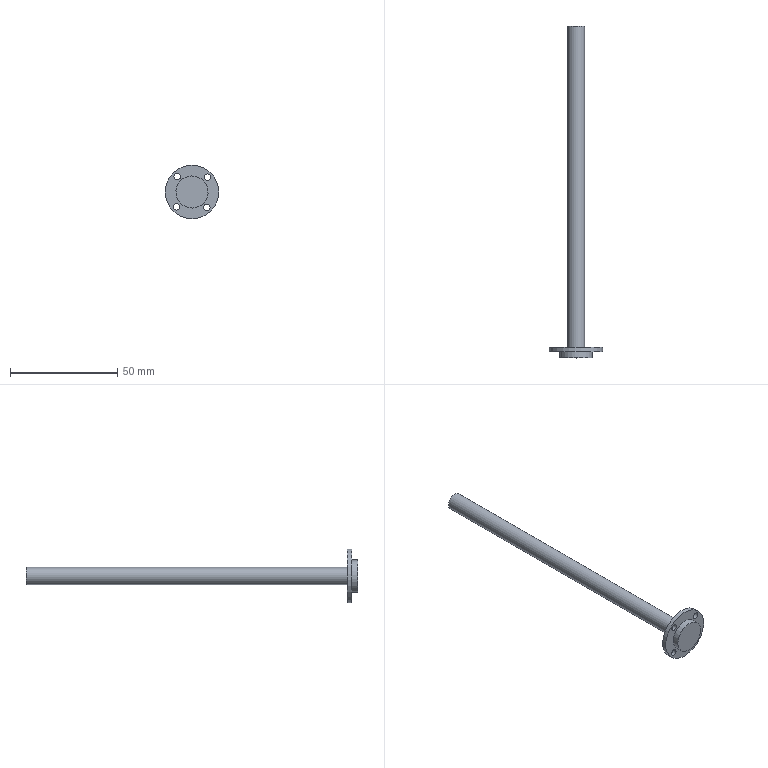Component | NX | GEAR_SHAFT_1 | 1 solid | 11 faces | box 25 x 155 x 25 mm | volume 8995 mm3 | cylinder 7 | plane 4 | commonest cylinder face diameters 3 x4 8 x1 25 x1 15 x1
STEP:
#1=CARTESIAN_POINT('',(0.,0.,0.));
#2=DIRECTION('',(0.,0.,1.));
#3=DIRECTION('',(1.,0.,0.));
#4=AXIS2_PLACEMENT_3D('',#1,#2,#3);
#5=CARTESIAN_POINT('',(-91.15,115.04,41.934));
#6=VERTEX_POINT('',#5);
#7=CARTESIAN_POINT('',(-88.383,115.04,39.046));
#8=DIRECTION('',(0.,-1.,0.));
#9=DIRECTION('',(-0.6919,0.,0.722));
#10=AXIS2_PLACEMENT_3D('',#7,#8,#9);
#11=CIRCLE('',#10,4.);
#12=CARTESIAN_POINT('',(-88.383,115.04,39.046));
#13=DIRECTION('',(0.,-1.,0.));
#14=DIRECTION('',(0.722,0.,0.6919));
#15=AXIS2_PLACEMENT_3D('',#12,#13,#14);
#16=CYLINDRICAL_SURFACE('',#15,4.);
#17=CARTESIAN_POINT('',(1.571,0.));
#18=DIRECTION('',(1.,0.));
#19=VECTOR('',#18,1.);
#20=LINE('',#17,#19);
#21=(GEOMETRIC_REPRESENTATION_CONTEXT(2)PARAMETRIC_REPRESENTATION_CONTEXT()REPRESENTATION_CONTEXT('',''));
#22=DEFINITIONAL_REPRESENTATION('',(#20),#21);
#23=PCURVE('',#16,#22);
#24=CARTESIAN_POINT('',(-88.383,115.04,39.046));
#25=DIRECTION('',(0.,-1.,0.));
#26=DIRECTION('',(0.722,0.,0.6919));
#27=AXIS2_PLACEMENT_3D('',#24,#25,#26);
#28=PLANE('',#27);
#29=CARTESIAN_POINT('',(0.,0.));
#30=DIRECTION('',(0.,1.));
#31=AXIS2_PLACEMENT_2D('',#29,#30);
#32=CIRCLE('',#31,4.);
#33=(GEOMETRIC_REPRESENTATION_CONTEXT(2)PARAMETRIC_REPRESENTATION_CONTEXT()REPRESENTATION_CONTEXT('',''));
#34=DEFINITIONAL_REPRESENTATION('',(#32),#33);
#35=PCURVE('',#28,#34);
#36=SURFACE_CURVE('',#11,(#23,#35),.PCURVE_S1.);
#37=EDGE_CURVE('',#6,#6,#36,.T.);
#38=ORIENTED_EDGE('',*,*,#37,.T.);
#39=CARTESIAN_POINT('',(-91.15,-34.96,41.934));
#40=VERTEX_POINT('',#39);
#41=CARTESIAN_POINT('',(-91.15,115.04,41.934));
#42=CARTESIAN_POINT('',(-91.15,-34.96,41.934));
#43=B_SPLINE_CURVE_WITH_KNOTS('',1,(#41,#42),.UNSPECIFIED.,.F.,.F.,(2,2),(0.,150.),.PIECEWISE_BEZIER_KNOTS.);
#44=CARTESIAN_POINT('',(7.854,0.));
#45=DIRECTION('',(0.,1.));
#46=VECTOR('',#45,1.);
#47=LINE('',#44,#46);
#48=(GEOMETRIC_REPRESENTATION_CONTEXT(2)PARAMETRIC_REPRESENTATION_CONTEXT()REPRESENTATION_CONTEXT('',''));
#49=DEFINITIONAL_REPRESENTATION('',(#47),#48);
#50=PCURVE('',#16,#49);
#51=CARTESIAN_POINT('',(1.571,0.));
#52=DIRECTION('',(0.,1.));
#53=VECTOR('',#52,1.);
#54=LINE('',#51,#53);
#55=(GEOMETRIC_REPRESENTATION_CONTEXT(2)PARAMETRIC_REPRESENTATION_CONTEXT()REPRESENTATION_CONTEXT('',''));
#56=DEFINITIONAL_REPRESENTATION('',(#54),#55);
#57=PCURVE('',#16,#56);
#58=SEAM_CURVE('',#43,(#50,#57),.PCURVE_S1.);
#59=EDGE_CURVE('',#6,#40,#58,.T.);
#60=ORIENTED_EDGE('',*,*,#59,.T.);
#61=CARTESIAN_POINT('',(-88.383,-34.96,39.046));
#62=DIRECTION('',(0.,-1.,0.));
#63=DIRECTION('',(-0.6919,0.,0.722));
#64=AXIS2_PLACEMENT_3D('',#61,#62,#63);
#65=CIRCLE('',#64,4.);
#66=CARTESIAN_POINT('',(1.571,150.));
#67=DIRECTION('',(1.,0.));
#68=VECTOR('',#67,1.);
#69=LINE('',#66,#68);
#70=(GEOMETRIC_REPRESENTATION_CONTEXT(2)PARAMETRIC_REPRESENTATION_CONTEXT()REPRESENTATION_CONTEXT('',''));
#71=DEFINITIONAL_REPRESENTATION('',(#69),#70);
#72=PCURVE('',#16,#71);
#73=CARTESIAN_POINT('',(-88.383,-34.96,39.046));
#74=DIRECTION('',(0.,-1.,0.));
#75=DIRECTION('',(0.722,0.,0.6919));
#76=AXIS2_PLACEMENT_3D('',#73,#74,#75);
#77=PLANE('',#76);
#78=CARTESIAN_POINT('',(0.,0.));
#79=DIRECTION('',(0.,1.));
#80=AXIS2_PLACEMENT_2D('',#78,#79);
#81=CIRCLE('',#80,4.);
#82=(GEOMETRIC_REPRESENTATION_CONTEXT(2)PARAMETRIC_REPRESENTATION_CONTEXT()REPRESENTATION_CONTEXT('',''));
#83=DEFINITIONAL_REPRESENTATION('',(#81),#82);
#84=PCURVE('',#77,#83);
#85=SURFACE_CURVE('',#65,(#72,#84),.PCURVE_S1.);
#86=EDGE_CURVE('',#40,#40,#85,.T.);
#87=ORIENTED_EDGE('',*,*,#86,.F.);
#88=ORIENTED_EDGE('',*,*,#59,.F.);
#89=EDGE_LOOP('',(#38,#60,#87,#88));
#90=FACE_BOUND('',#89,.T.);
#91=ADVANCED_FACE('',(#90),#16,.T.);
#92=ORIENTED_EDGE('',*,*,#37,.F.);
#93=EDGE_LOOP('',(#92));
#94=FACE_BOUND('',#93,.T.);
#95=ADVANCED_FACE('',(#94),#28,.F.);
#96=CARTESIAN_POINT('',(-97.032,-36.96,48.071));
#97=VERTEX_POINT('',#96);
#98=CARTESIAN_POINT('',(-88.383,-36.96,39.046));
#99=DIRECTION('',(0.,1.,0.));
#100=DIRECTION('',(-0.6919,0.,0.722));
#101=AXIS2_PLACEMENT_3D('',#98,#99,#100);
#102=CIRCLE('',#101,12.5);
#103=CARTESIAN_POINT('',(-88.383,-36.96,39.046));
#104=DIRECTION('',(0.,1.,0.));
#105=DIRECTION('',(-0.722,0.,-0.6919));
#106=AXIS2_PLACEMENT_3D('',#103,#104,#105);
#107=CYLINDRICAL_SURFACE('',#106,12.5);
#108=CARTESIAN_POINT('',(1.571,0.));
#109=DIRECTION('',(1.,0.));
#110=VECTOR('',#109,1.);
#111=LINE('',#108,#110);
#112=(GEOMETRIC_REPRESENTATION_CONTEXT(2)PARAMETRIC_REPRESENTATION_CONTEXT()REPRESENTATION_CONTEXT('',''));
#113=DEFINITIONAL_REPRESENTATION('',(#111),#112);
#114=PCURVE('',#107,#113);
#115=CARTESIAN_POINT('',(-88.383,-36.96,39.046));
#116=DIRECTION('',(0.,-1.,0.));
#117=DIRECTION('',(0.722,0.,0.6919));
#118=AXIS2_PLACEMENT_3D('',#115,#116,#117);
#119=PLANE('',#118);
#120=CARTESIAN_POINT('',(0.,12.5));
#121=CARTESIAN_POINT('',(21.651,12.5));
#122=CARTESIAN_POINT('',(10.825,-6.25));
#123=CARTESIAN_POINT('',(-0.,-25.));
#124=CARTESIAN_POINT('',(-10.825,-6.25));
#125=CARTESIAN_POINT('',(-21.651,12.5));
#126=CARTESIAN_POINT('',(0.,12.5));
#127=(BOUNDED_CURVE()B_SPLINE_CURVE(2,(#120,#121,#122,#123,#124,#125,#126),.UNSPECIFIED.,.T.,.F.)B_SPLINE_CURVE_WITH_KNOTS((1,2,2,2,2,1),(-2.094,0.,2.094,4.189,6.283,8.378),.UNSPECIFIED.)CURVE()GEOMETRIC_REPRESENTATION_ITEM()RATIONAL_B_SPLINE_CURVE((1.,0.5,1.,0.5,1.,0.5,1.))REPRESENTATION_ITEM(''));
#128=(GEOMETRIC_REPRESENTATION_CONTEXT(2)PARAMETRIC_REPRESENTATION_CONTEXT()REPRESENTATION_CONTEXT('',''));
#129=DEFINITIONAL_REPRESENTATION('',(#127),#128);
#130=PCURVE('',#119,#129);
#131=SURFACE_CURVE('',#102,(#114,#130),.PCURVE_S1.);
#132=EDGE_CURVE('',#97,#97,#131,.T.);
#133=ORIENTED_EDGE('',*,*,#132,.T.);
#134=CARTESIAN_POINT('',(-97.032,-34.96,48.071));
#135=VERTEX_POINT('',#134);
#136=CARTESIAN_POINT('',(-97.032,-36.96,48.071));
#137=CARTESIAN_POINT('',(-97.032,-34.96,48.071));
#138=B_SPLINE_CURVE_WITH_KNOTS('',1,(#136,#137),.UNSPECIFIED.,.F.,.F.,(2,2),(0.,2.),.PIECEWISE_BEZIER_KNOTS.);
#139=CARTESIAN_POINT('',(7.854,0.));
#140=DIRECTION('',(0.,1.));
#141=VECTOR('',#140,1.);
#142=LINE('',#139,#141);
#143=(GEOMETRIC_REPRESENTATION_CONTEXT(2)PARAMETRIC_REPRESENTATION_CONTEXT()REPRESENTATION_CONTEXT('',''));
#144=DEFINITIONAL_REPRESENTATION('',(#142),#143);
#145=PCURVE('',#107,#144);
#146=CARTESIAN_POINT('',(1.571,0.));
#147=DIRECTION('',(0.,1.));
#148=VECTOR('',#147,1.);
#149=LINE('',#146,#148);
#150=(GEOMETRIC_REPRESENTATION_CONTEXT(2)PARAMETRIC_REPRESENTATION_CONTEXT()REPRESENTATION_CONTEXT('',''));
#151=DEFINITIONAL_REPRESENTATION('',(#149),#150);
#152=PCURVE('',#107,#151);
#153=SEAM_CURVE('',#138,(#145,#152),.PCURVE_S1.);
#154=EDGE_CURVE('',#97,#135,#153,.T.);
#155=ORIENTED_EDGE('',*,*,#154,.T.);
#156=CARTESIAN_POINT('',(-88.383,-34.96,39.046));
#157=DIRECTION('',(0.,1.,0.));
#158=DIRECTION('',(-0.6919,0.,0.722));
#159=AXIS2_PLACEMENT_3D('',#156,#157,#158);
#160=CIRCLE('',#159,12.5);
#161=CARTESIAN_POINT('',(1.571,2.));
#162=DIRECTION('',(1.,0.));
#163=VECTOR('',#162,1.);
#164=LINE('',#161,#163);
#165=(GEOMETRIC_REPRESENTATION_CONTEXT(2)PARAMETRIC_REPRESENTATION_CONTEXT()REPRESENTATION_CONTEXT('',''));
#166=DEFINITIONAL_REPRESENTATION('',(#164),#165);
#167=PCURVE('',#107,#166);
#168=CARTESIAN_POINT('',(0.,12.5));
#169=CARTESIAN_POINT('',(21.651,12.5));
#170=CARTESIAN_POINT('',(10.825,-6.25));
#171=CARTESIAN_POINT('',(-0.,-25.));
#172=CARTESIAN_POINT('',(-10.825,-6.25));
#173=CARTESIAN_POINT('',(-21.651,12.5));
#174=CARTESIAN_POINT('',(0.,12.5));
#175=(BOUNDED_CURVE()B_SPLINE_CURVE(2,(#168,#169,#170,#171,#172,#173,#174),.UNSPECIFIED.,.T.,.F.)B_SPLINE_CURVE_WITH_KNOTS((1,2,2,2,2,1),(-2.094,0.,2.094,4.189,6.283,8.378),.UNSPECIFIED.)CURVE()GEOMETRIC_REPRESENTATION_ITEM()RATIONAL_B_SPLINE_CURVE((1.,0.5,1.,0.5,1.,0.5,1.))REPRESENTATION_ITEM(''));
#176=(GEOMETRIC_REPRESENTATION_CONTEXT(2)PARAMETRIC_REPRESENTATION_CONTEXT()REPRESENTATION_CONTEXT('',''));
#177=DEFINITIONAL_REPRESENTATION('',(#175),#176);
#178=PCURVE('',#77,#177);
#179=SURFACE_CURVE('',#160,(#167,#178),.PCURVE_S1.);
#180=EDGE_CURVE('',#135,#135,#179,.T.);
#181=ORIENTED_EDGE('',*,*,#180,.F.);
#182=ORIENTED_EDGE('',*,*,#154,.F.);
#183=EDGE_LOOP('',(#133,#155,#181,#182));
#184=FACE_BOUND('',#183,.T.);
#185=ADVANCED_FACE('',(#184),#107,.T.);
#186=CARTESIAN_POINT('',(-96.685,-36.96,31.089));
#187=VERTEX_POINT('',#186);
#188=CARTESIAN_POINT('',(-94.519,-36.96,33.165));
#189=VERTEX_POINT('',#188);
#190=CARTESIAN_POINT('',(-95.602,-36.96,32.127));
#191=DIRECTION('',(0.,1.,0.));
#192=DIRECTION('',(-0.722,0.,-0.6919));
#193=AXIS2_PLACEMENT_3D('',#190,#191,#192);
#194=CIRCLE('',#193,1.5);
#195=CARTESIAN_POINT('',(-11.5,0.));
#196=CARTESIAN_POINT('',(-11.5,2.598));
#197=CARTESIAN_POINT('',(-9.25,1.299));
#198=CARTESIAN_POINT('',(-7.,0.));
#199=CARTESIAN_POINT('',(-9.25,-1.299));
#200=CARTESIAN_POINT('',(-11.5,-2.598));
#201=CARTESIAN_POINT('',(-11.5,0.));
#202=(BOUNDED_CURVE()B_SPLINE_CURVE(2,(#195,#196,#197,#198,#199,#200,#201),.UNSPECIFIED.,.T.,.F.)B_SPLINE_CURVE_WITH_KNOTS((1,2,2,2,2,1),(-2.094,0.,2.094,4.189,6.283,8.378),.UNSPECIFIED.)CURVE()GEOMETRIC_REPRESENTATION_ITEM()RATIONAL_B_SPLINE_CURVE((1.,0.5,1.,0.5,1.,0.5,1.))REPRESENTATION_ITEM(''));
#203=(GEOMETRIC_REPRESENTATION_CONTEXT(2)PARAMETRIC_REPRESENTATION_CONTEXT()REPRESENTATION_CONTEXT('',''));
#204=DEFINITIONAL_REPRESENTATION('',(#202),#203);
#205=PCURVE('',#119,#204);
#206=CARTESIAN_POINT('',(-95.602,163.04,32.127));
#207=DIRECTION('',(0.,-1.,0.));
#208=DIRECTION('',(0.722,0.,0.6919));
#209=AXIS2_PLACEMENT_3D('',#206,#207,#208);
#210=CYLINDRICAL_SURFACE('',#209,1.5);
#211=CARTESIAN_POINT('',(3.142,200.));
#212=DIRECTION('',(-1.,0.));
#213=VECTOR('',#212,1.);
#214=LINE('',#211,#213);
#215=(GEOMETRIC_REPRESENTATION_CONTEXT(2)PARAMETRIC_REPRESENTATION_CONTEXT()REPRESENTATION_CONTEXT('',''));
#216=DEFINITIONAL_REPRESENTATION('',(#214),#215);
#217=PCURVE('',#210,#216);
#218=SURFACE_CURVE('',#194,(#205,#217),.PCURVE_S1.);
#219=EDGE_CURVE('',#187,#189,#218,.T.);
#220=ORIENTED_EDGE('',*,*,#219,.T.);
#221=CARTESIAN_POINT('',(-95.602,-36.96,32.127));
#222=DIRECTION('',(0.,1.,0.));
#223=DIRECTION('',(-0.722,0.,-0.6919));
#224=AXIS2_PLACEMENT_3D('',#221,#222,#223);
#225=CIRCLE('',#224,1.5);
#226=CARTESIAN_POINT('',(-11.5,0.));
#227=CARTESIAN_POINT('',(-11.5,2.598));
#228=CARTESIAN_POINT('',(-9.25,1.299));
#229=CARTESIAN_POINT('',(-7.,0.));
#230=CARTESIAN_POINT('',(-9.25,-1.299));
#231=CARTESIAN_POINT('',(-11.5,-2.598));
#232=CARTESIAN_POINT('',(-11.5,0.));
#233=(BOUNDED_CURVE()B_SPLINE_CURVE(2,(#226,#227,#228,#229,#230,#231,#232),.UNSPECIFIED.,.T.,.F.)B_SPLINE_CURVE_WITH_KNOTS((1,2,2,2,2,1),(-2.094,0.,2.094,4.189,6.283,8.378),.UNSPECIFIED.)CURVE()GEOMETRIC_REPRESENTATION_ITEM()RATIONAL_B_SPLINE_CURVE((1.,0.5,1.,0.5,1.,0.5,1.))REPRESENTATION_ITEM(''));
#234=(GEOMETRIC_REPRESENTATION_CONTEXT(2)PARAMETRIC_REPRESENTATION_CONTEXT()REPRESENTATION_CONTEXT('',''));
#235=DEFINITIONAL_REPRESENTATION('',(#233),#234);
#236=PCURVE('',#119,#235);
#237=CARTESIAN_POINT('',(9.425,200.));
#238=DIRECTION('',(-1.,0.));
#239=VECTOR('',#238,1.);
#240=LINE('',#237,#239);
#241=(GEOMETRIC_REPRESENTATION_CONTEXT(2)PARAMETRIC_REPRESENTATION_CONTEXT()REPRESENTATION_CONTEXT('',''));
#242=DEFINITIONAL_REPRESENTATION('',(#240),#241);
#243=PCURVE('',#210,#242);
#244=SURFACE_CURVE('',#225,(#236,#243),.PCURVE_S1.);
#245=EDGE_CURVE('',#189,#187,#244,.T.);
#246=ORIENTED_EDGE('',*,*,#245,.T.);
#247=EDGE_LOOP('',(#220,#246));
#248=FACE_BOUND('',#247,.T.);
#249=CARTESIAN_POINT('',(-80.426,-36.96,30.744));
#250=VERTEX_POINT('',#249);
#251=CARTESIAN_POINT('',(-80.381,-36.96,32.865));
#252=VERTEX_POINT('',#251);
#253=CARTESIAN_POINT('',(-81.463,-36.96,31.827));
#254=DIRECTION('',(0.,-1.,0.));
#255=DIRECTION('',(0.6919,0.,-0.722));
#256=AXIS2_PLACEMENT_3D('',#253,#254,#255);
#257=CIRCLE('',#256,1.5);
#258=CARTESIAN_POINT('',(-0.,-10.));
#259=DIRECTION('',(-0.,-1.));
#260=AXIS2_PLACEMENT_2D('',#258,#259);
#261=CIRCLE('',#260,1.5);
#262=(GEOMETRIC_REPRESENTATION_CONTEXT(2)PARAMETRIC_REPRESENTATION_CONTEXT()REPRESENTATION_CONTEXT('',''));
#263=DEFINITIONAL_REPRESENTATION('',(#261),#262);
#264=PCURVE('',#119,#263);
#265=CARTESIAN_POINT('',(-81.463,163.04,31.827));
#266=DIRECTION('',(0.,-1.,0.));
#267=DIRECTION('',(0.722,0.,0.6919));
#268=AXIS2_PLACEMENT_3D('',#265,#266,#267);
#269=CYLINDRICAL_SURFACE('',#268,1.5);
#270=CARTESIAN_POINT('',(4.712,200.));
#271=DIRECTION('',(1.,0.));
#272=VECTOR('',#271,1.);
#273=LINE('',#270,#272);
#274=(GEOMETRIC_REPRESENTATION_CONTEXT(2)PARAMETRIC_REPRESENTATION_CONTEXT()REPRESENTATION_CONTEXT('',''));
#275=DEFINITIONAL_REPRESENTATION('',(#273),#274);
#276=PCURVE('',#269,#275);
#277=SURFACE_CURVE('',#257,(#264,#276),.PCURVE_S1.);
#278=EDGE_CURVE('',#250,#252,#277,.T.);
#279=ORIENTED_EDGE('',*,*,#278,.F.);
#280=CARTESIAN_POINT('',(-81.463,-36.96,31.827));
#281=DIRECTION('',(0.,-1.,0.));
#282=DIRECTION('',(0.6919,0.,-0.722));
#283=AXIS2_PLACEMENT_3D('',#280,#281,#282);
#284=CIRCLE('',#283,1.5);
#285=CARTESIAN_POINT('',(-0.,-10.));
#286=DIRECTION('',(-0.,-1.));
#287=AXIS2_PLACEMENT_2D('',#285,#286);
#288=CIRCLE('',#287,1.5);
#289=(GEOMETRIC_REPRESENTATION_CONTEXT(2)PARAMETRIC_REPRESENTATION_CONTEXT()REPRESENTATION_CONTEXT('',''));
#290=DEFINITIONAL_REPRESENTATION('',(#288),#289);
#291=PCURVE('',#119,#290);
#292=CARTESIAN_POINT('',(-1.571,200.));
#293=DIRECTION('',(1.,0.));
#294=VECTOR('',#293,1.);
#295=LINE('',#292,#294);
#296=(GEOMETRIC_REPRESENTATION_CONTEXT(2)PARAMETRIC_REPRESENTATION_CONTEXT()REPRESENTATION_CONTEXT('',''));
#297=DEFINITIONAL_REPRESENTATION('',(#295),#296);
#298=PCURVE('',#269,#297);
#299=SURFACE_CURVE('',#284,(#291,#298),.PCURVE_S1.);
#300=EDGE_CURVE('',#252,#250,#299,.T.);
#301=ORIENTED_EDGE('',*,*,#300,.F.);
#302=EDGE_LOOP('',(#279,#301));
#303=FACE_BOUND('',#302,.T.);
#304=CARTESIAN_POINT('',(-80.08,-36.96,47.004));
#305=VERTEX_POINT('',#304);
#306=CARTESIAN_POINT('',(-81.163,-36.96,45.966));
#307=DIRECTION('',(0.,-1.,0.));
#308=DIRECTION('',(0.722,0.,0.6919));
#309=AXIS2_PLACEMENT_3D('',#306,#307,#308);
#310=CIRCLE('',#309,1.5);
#311=CARTESIAN_POINT('',(10.,0.));
#312=DIRECTION('',(1.,-0.));
#313=AXIS2_PLACEMENT_2D('',#311,#312);
#314=CIRCLE('',#313,1.5);
#315=(GEOMETRIC_REPRESENTATION_CONTEXT(2)PARAMETRIC_REPRESENTATION_CONTEXT()REPRESENTATION_CONTEXT('',''));
#316=DEFINITIONAL_REPRESENTATION('',(#314),#315);
#317=PCURVE('',#119,#316);
#318=CARTESIAN_POINT('',(-81.163,163.04,45.966));
#319=DIRECTION('',(0.,-1.,0.));
#320=DIRECTION('',(0.722,0.,0.6919));
#321=AXIS2_PLACEMENT_3D('',#318,#319,#320);
#322=CYLINDRICAL_SURFACE('',#321,1.5);
#323=CARTESIAN_POINT('',(0.,200.));
#324=DIRECTION('',(1.,0.));
#325=VECTOR('',#324,1.);
#326=LINE('',#323,#325);
#327=(GEOMETRIC_REPRESENTATION_CONTEXT(2)PARAMETRIC_REPRESENTATION_CONTEXT()REPRESENTATION_CONTEXT('',''));
#328=DEFINITIONAL_REPRESENTATION('',(#326),#327);
#329=PCURVE('',#322,#328);
#330=SURFACE_CURVE('',#310,(#317,#329),.PCURVE_S1.);
#331=EDGE_CURVE('',#305,#305,#330,.T.);
#332=ORIENTED_EDGE('',*,*,#331,.F.);
#333=EDGE_LOOP('',(#332));
#334=FACE_BOUND('',#333,.T.);
#335=CARTESIAN_POINT('',(-96.34,-36.96,47.349));
#336=VERTEX_POINT('',#335);
#337=CARTESIAN_POINT('',(-94.219,-36.96,47.304));
#338=VERTEX_POINT('',#337);
#339=CARTESIAN_POINT('',(-95.302,-36.96,46.266));
#340=DIRECTION('',(0.,-1.,0.));
#341=DIRECTION('',(-0.6919,0.,0.722));
#342=AXIS2_PLACEMENT_3D('',#339,#340,#341);
#343=CIRCLE('',#342,1.5);
#344=CARTESIAN_POINT('',(-0.,10.));
#345=DIRECTION('',(0.,1.));
#346=AXIS2_PLACEMENT_2D('',#344,#345);
#347=CIRCLE('',#346,1.5);
#348=(GEOMETRIC_REPRESENTATION_CONTEXT(2)PARAMETRIC_REPRESENTATION_CONTEXT()REPRESENTATION_CONTEXT('',''));
#349=DEFINITIONAL_REPRESENTATION('',(#347),#348);
#350=PCURVE('',#119,#349);
#351=CARTESIAN_POINT('',(-95.302,163.04,46.266));
#352=DIRECTION('',(0.,-1.,0.));
#353=DIRECTION('',(0.722,0.,0.6919));
#354=AXIS2_PLACEMENT_3D('',#351,#352,#353);
#355=CYLINDRICAL_SURFACE('',#354,1.5);
#356=CARTESIAN_POINT('',(1.571,200.));
#357=DIRECTION('',(1.,0.));
#358=VECTOR('',#357,1.);
#359=LINE('',#356,#358);
#360=(GEOMETRIC_REPRESENTATION_CONTEXT(2)PARAMETRIC_REPRESENTATION_CONTEXT()REPRESENTATION_CONTEXT('',''));
#361=DEFINITIONAL_REPRESENTATION('',(#359),#360);
#362=PCURVE('',#355,#361);
#363=SURFACE_CURVE('',#343,(#350,#362),.PCURVE_S1.);
#364=EDGE_CURVE('',#336,#338,#363,.T.);
#365=ORIENTED_EDGE('',*,*,#364,.F.);
#366=CARTESIAN_POINT('',(-95.302,-36.96,46.266));
#367=DIRECTION('',(0.,-1.,0.));
#368=DIRECTION('',(-0.6919,0.,0.722));
#369=AXIS2_PLACEMENT_3D('',#366,#367,#368);
#370=CIRCLE('',#369,1.5);
#371=CARTESIAN_POINT('',(-0.,10.));
#372=DIRECTION('',(0.,1.));
#373=AXIS2_PLACEMENT_2D('',#371,#372);
#374=CIRCLE('',#373,1.5);
#375=(GEOMETRIC_REPRESENTATION_CONTEXT(2)PARAMETRIC_REPRESENTATION_CONTEXT()REPRESENTATION_CONTEXT('',''));
#376=DEFINITIONAL_REPRESENTATION('',(#374),#375);
#377=PCURVE('',#119,#376);
#378=CARTESIAN_POINT('',(-4.712,200.));
#379=DIRECTION('',(1.,0.));
#380=VECTOR('',#379,1.);
#381=LINE('',#378,#380);
#382=(GEOMETRIC_REPRESENTATION_CONTEXT(2)PARAMETRIC_REPRESENTATION_CONTEXT()REPRESENTATION_CONTEXT('',''));
#383=DEFINITIONAL_REPRESENTATION('',(#381),#382);
#384=PCURVE('',#355,#383);
#385=SURFACE_CURVE('',#370,(#377,#384),.PCURVE_S1.);
#386=EDGE_CURVE('',#338,#336,#385,.T.);
#387=ORIENTED_EDGE('',*,*,#386,.F.);
#388=EDGE_LOOP('',(#365,#387));
#389=FACE_BOUND('',#388,.T.);
#390=CARTESIAN_POINT('',(-93.572,-36.96,44.461));
#391=VERTEX_POINT('',#390);
#392=CARTESIAN_POINT('',(-88.383,-36.96,39.046));
#393=DIRECTION('',(0.,-1.,0.));
#394=DIRECTION('',(-0.6919,0.,0.722));
#395=AXIS2_PLACEMENT_3D('',#392,#393,#394);
#396=CIRCLE('',#395,7.5);
#397=CARTESIAN_POINT('',(0.,0.));
#398=DIRECTION('',(0.,1.));
#399=AXIS2_PLACEMENT_2D('',#397,#398);
#400=CIRCLE('',#399,7.5);
#401=(GEOMETRIC_REPRESENTATION_CONTEXT(2)PARAMETRIC_REPRESENTATION_CONTEXT()REPRESENTATION_CONTEXT('',''));
#402=DEFINITIONAL_REPRESENTATION('',(#400),#401);
#403=PCURVE('',#119,#402);
#404=CARTESIAN_POINT('',(-88.383,-39.96,39.046));
#405=DIRECTION('',(0.,1.,0.));
#406=DIRECTION('',(-0.722,0.,-0.6919));
#407=AXIS2_PLACEMENT_3D('',#404,#405,#406);
#408=CYLINDRICAL_SURFACE('',#407,7.5);
#409=CARTESIAN_POINT('',(7.854,3.));
#410=DIRECTION('',(-1.,0.));
#411=VECTOR('',#410,1.);
#412=LINE('',#409,#411);
#413=(GEOMETRIC_REPRESENTATION_CONTEXT(2)PARAMETRIC_REPRESENTATION_CONTEXT()REPRESENTATION_CONTEXT('',''));
#414=DEFINITIONAL_REPRESENTATION('',(#412),#413);
#415=PCURVE('',#408,#414);
#416=SURFACE_CURVE('',#396,(#403,#415),.PCURVE_S1.);
#417=EDGE_CURVE('',#391,#391,#416,.T.);
#418=ORIENTED_EDGE('',*,*,#417,.F.);
#419=EDGE_LOOP('',(#418));
#420=FACE_BOUND('',#419,.T.);
#421=ORIENTED_EDGE('',*,*,#132,.F.);
#422=EDGE_LOOP('',(#421));
#423=FACE_BOUND('',#422,.T.);
#424=ADVANCED_FACE('',(#248,#303,#334,#389,#420,#423),#119,.T.);
#425=CARTESIAN_POINT('',(-94.519,-34.96,33.165));
#426=VERTEX_POINT('',#425);
#427=CARTESIAN_POINT('',(-95.602,-34.96,32.127));
#428=DIRECTION('',(0.,1.,0.));
#429=DIRECTION('',(0.722,0.,0.6919));
#430=AXIS2_PLACEMENT_3D('',#427,#428,#429);
#431=CIRCLE('',#430,1.5);
#432=CARTESIAN_POINT('',(-8.5,0.));
#433=CARTESIAN_POINT('',(-8.5,-2.598));
#434=CARTESIAN_POINT('',(-10.75,-1.299));
#435=CARTESIAN_POINT('',(-13.,0.));
#436=CARTESIAN_POINT('',(-10.75,1.299));
#437=CARTESIAN_POINT('',(-8.5,2.598));
#438=CARTESIAN_POINT('',(-8.5,0.));
#439=(BOUNDED_CURVE()B_SPLINE_CURVE(2,(#432,#433,#434,#435,#436,#437,#438),.UNSPECIFIED.,.T.,.F.)B_SPLINE_CURVE_WITH_KNOTS((1,2,2,2,2,1),(-2.094,0.,2.094,4.189,6.283,8.378),.UNSPECIFIED.)CURVE()GEOMETRIC_REPRESENTATION_ITEM()RATIONAL_B_SPLINE_CURVE((1.,0.5,1.,0.5,1.,0.5,1.))REPRESENTATION_ITEM(''));
#440=(GEOMETRIC_REPRESENTATION_CONTEXT(2)PARAMETRIC_REPRESENTATION_CONTEXT()REPRESENTATION_CONTEXT('',''));
#441=DEFINITIONAL_REPRESENTATION('',(#439),#440);
#442=PCURVE('',#77,#441);
#443=CARTESIAN_POINT('',(6.283,198.));
#444=DIRECTION('',(-1.,0.));
#445=VECTOR('',#444,1.);
#446=LINE('',#443,#445);
#447=(GEOMETRIC_REPRESENTATION_CONTEXT(2)PARAMETRIC_REPRESENTATION_CONTEXT()REPRESENTATION_CONTEXT('',''));
#448=DEFINITIONAL_REPRESENTATION('',(#446),#447);
#449=PCURVE('',#210,#448);
#450=SURFACE_CURVE('',#431,(#442,#449),.PCURVE_S1.);
#451=EDGE_CURVE('',#426,#426,#450,.T.);
#452=ORIENTED_EDGE('',*,*,#451,.F.);
#453=EDGE_LOOP('',(#452));
#454=FACE_BOUND('',#453,.T.);
#455=CARTESIAN_POINT('',(-80.381,-34.96,32.865));
#456=VERTEX_POINT('',#455);
#457=CARTESIAN_POINT('',(-81.463,-34.96,31.827));
#458=DIRECTION('',(0.,-1.,0.));
#459=DIRECTION('',(0.722,0.,0.6919));
#460=AXIS2_PLACEMENT_3D('',#457,#458,#459);
#461=CIRCLE('',#460,1.5);
#462=CARTESIAN_POINT('',(-0.,-10.));
#463=DIRECTION('',(1.,-0.));
#464=AXIS2_PLACEMENT_2D('',#462,#463);
#465=CIRCLE('',#464,1.5);
#466=(GEOMETRIC_REPRESENTATION_CONTEXT(2)PARAMETRIC_REPRESENTATION_CONTEXT()REPRESENTATION_CONTEXT('',''));
#467=DEFINITIONAL_REPRESENTATION('',(#465),#466);
#468=PCURVE('',#77,#467);
#469=CARTESIAN_POINT('',(0.,198.));
#470=DIRECTION('',(1.,0.));
#471=VECTOR('',#470,1.);
#472=LINE('',#469,#471);
#473=(GEOMETRIC_REPRESENTATION_CONTEXT(2)PARAMETRIC_REPRESENTATION_CONTEXT()REPRESENTATION_CONTEXT('',''));
#474=DEFINITIONAL_REPRESENTATION('',(#472),#473);
#475=PCURVE('',#269,#474);
#476=SURFACE_CURVE('',#461,(#468,#475),.PCURVE_S1.);
#477=EDGE_CURVE('',#456,#456,#476,.T.);
#478=ORIENTED_EDGE('',*,*,#477,.T.);
#479=EDGE_LOOP('',(#478));
#480=FACE_BOUND('',#479,.T.);
#481=CARTESIAN_POINT('',(-80.08,-34.96,47.004));
#482=VERTEX_POINT('',#481);
#483=CARTESIAN_POINT('',(-81.163,-34.96,45.966));
#484=DIRECTION('',(0.,-1.,0.));
#485=DIRECTION('',(0.722,0.,0.6919));
#486=AXIS2_PLACEMENT_3D('',#483,#484,#485);
#487=CIRCLE('',#486,1.5);
#488=CARTESIAN_POINT('',(10.,0.));
#489=DIRECTION('',(1.,-0.));
#490=AXIS2_PLACEMENT_2D('',#488,#489);
#491=CIRCLE('',#490,1.5);
#492=(GEOMETRIC_REPRESENTATION_CONTEXT(2)PARAMETRIC_REPRESENTATION_CONTEXT()REPRESENTATION_CONTEXT('',''));
#493=DEFINITIONAL_REPRESENTATION('',(#491),#492);
#494=PCURVE('',#77,#493);
#495=CARTESIAN_POINT('',(0.,198.));
#496=DIRECTION('',(1.,0.));
#497=VECTOR('',#496,1.);
#498=LINE('',#495,#497);
#499=(GEOMETRIC_REPRESENTATION_CONTEXT(2)PARAMETRIC_REPRESENTATION_CONTEXT()REPRESENTATION_CONTEXT('',''));
#500=DEFINITIONAL_REPRESENTATION('',(#498),#499);
#501=PCURVE('',#322,#500);
#502=SURFACE_CURVE('',#487,(#494,#501),.PCURVE_S1.);
#503=EDGE_CURVE('',#482,#482,#502,.T.);
#504=ORIENTED_EDGE('',*,*,#503,.T.);
#505=EDGE_LOOP('',(#504));
#506=FACE_BOUND('',#505,.T.);
#507=CARTESIAN_POINT('',(-94.219,-34.96,47.304));
#508=VERTEX_POINT('',#507);
#509=CARTESIAN_POINT('',(-95.302,-34.96,46.266));
#510=DIRECTION('',(0.,-1.,0.));
#511=DIRECTION('',(0.722,0.,0.6919));
#512=AXIS2_PLACEMENT_3D('',#509,#510,#511);
#513=CIRCLE('',#512,1.5);
#514=CARTESIAN_POINT('',(-0.,10.));
#515=DIRECTION('',(1.,-0.));
#516=AXIS2_PLACEMENT_2D('',#514,#515);
#517=CIRCLE('',#516,1.5);
#518=(GEOMETRIC_REPRESENTATION_CONTEXT(2)PARAMETRIC_REPRESENTATION_CONTEXT()REPRESENTATION_CONTEXT('',''));
#519=DEFINITIONAL_REPRESENTATION('',(#517),#518);
#520=PCURVE('',#77,#519);
#521=CARTESIAN_POINT('',(0.,198.));
#522=DIRECTION('',(1.,0.));
#523=VECTOR('',#522,1.);
#524=LINE('',#521,#523);
#525=(GEOMETRIC_REPRESENTATION_CONTEXT(2)PARAMETRIC_REPRESENTATION_CONTEXT()REPRESENTATION_CONTEXT('',''));
#526=DEFINITIONAL_REPRESENTATION('',(#524),#525);
#527=PCURVE('',#355,#526);
#528=SURFACE_CURVE('',#513,(#520,#527),.PCURVE_S1.);
#529=EDGE_CURVE('',#508,#508,#528,.T.);
#530=ORIENTED_EDGE('',*,*,#529,.T.);
#531=EDGE_LOOP('',(#530));
#532=FACE_BOUND('',#531,.T.);
#533=ORIENTED_EDGE('',*,*,#86,.T.);
#534=EDGE_LOOP('',(#533));
#535=FACE_BOUND('',#534,.T.);
#536=ORIENTED_EDGE('',*,*,#180,.T.);
#537=EDGE_LOOP('',(#536));
#538=FACE_BOUND('',#537,.T.);
#539=ADVANCED_FACE('',(#454,#480,#506,#532,#535,#538),#77,.F.);
#540=CARTESIAN_POINT('',(-93.572,-39.96,44.461));
#541=VERTEX_POINT('',#540);
#542=CARTESIAN_POINT('',(-88.383,-39.96,39.046));
#543=DIRECTION('',(0.,-1.,0.));
#544=DIRECTION('',(-0.6919,0.,0.722));
#545=AXIS2_PLACEMENT_3D('',#542,#543,#544);
#546=CIRCLE('',#545,7.5);
#547=CARTESIAN_POINT('',(7.854,0.));
#548=DIRECTION('',(-1.,0.));
#549=VECTOR('',#548,1.);
#550=LINE('',#547,#549);
#551=(GEOMETRIC_REPRESENTATION_CONTEXT(2)PARAMETRIC_REPRESENTATION_CONTEXT()REPRESENTATION_CONTEXT('',''));
#552=DEFINITIONAL_REPRESENTATION('',(#550),#551);
#553=PCURVE('',#408,#552);
#554=CARTESIAN_POINT('',(-88.383,-39.96,39.046));
#555=DIRECTION('',(0.,-1.,0.));
#556=DIRECTION('',(0.722,0.,0.6919));
#557=AXIS2_PLACEMENT_3D('',#554,#555,#556);
#558=PLANE('',#557);
#559=CARTESIAN_POINT('',(0.,0.));
#560=DIRECTION('',(0.,1.));
#561=AXIS2_PLACEMENT_2D('',#559,#560);
#562=CIRCLE('',#561,7.5);
#563=(GEOMETRIC_REPRESENTATION_CONTEXT(2)PARAMETRIC_REPRESENTATION_CONTEXT()REPRESENTATION_CONTEXT('',''));
#564=DEFINITIONAL_REPRESENTATION('',(#562),#563);
#565=PCURVE('',#558,#564);
#566=SURFACE_CURVE('',#546,(#553,#565),.PCURVE_S1.);
#567=EDGE_CURVE('',#541,#541,#566,.T.);
#568=ORIENTED_EDGE('',*,*,#567,.F.);
#569=CARTESIAN_POINT('',(-93.572,-39.96,44.461));
#570=CARTESIAN_POINT('',(-93.572,-36.96,44.461));
#571=B_SPLINE_CURVE_WITH_KNOTS('',1,(#569,#570),.UNSPECIFIED.,.F.,.F.,(2,2),(0.,3.),.PIECEWISE_BEZIER_KNOTS.);
#572=CARTESIAN_POINT('',(7.854,0.));
#573=DIRECTION('',(0.,1.));
#574=VECTOR('',#573,1.);
#575=LINE('',#572,#574);
#576=(GEOMETRIC_REPRESENTATION_CONTEXT(2)PARAMETRIC_REPRESENTATION_CONTEXT()REPRESENTATION_CONTEXT('',''));
#577=DEFINITIONAL_REPRESENTATION('',(#575),#576);
#578=PCURVE('',#408,#577);
#579=CARTESIAN_POINT('',(1.571,0.));
#580=DIRECTION('',(0.,1.));
#581=VECTOR('',#580,1.);
#582=LINE('',#579,#581);
#583=(GEOMETRIC_REPRESENTATION_CONTEXT(2)PARAMETRIC_REPRESENTATION_CONTEXT()REPRESENTATION_CONTEXT('',''));
#584=DEFINITIONAL_REPRESENTATION('',(#582),#583);
#585=PCURVE('',#408,#584);
#586=SEAM_CURVE('',#571,(#578,#585),.PCURVE_S1.);
#587=EDGE_CURVE('',#541,#391,#586,.T.);
#588=ORIENTED_EDGE('',*,*,#587,.T.);
#589=ORIENTED_EDGE('',*,*,#417,.T.);
#590=ORIENTED_EDGE('',*,*,#587,.F.);
#591=EDGE_LOOP('',(#568,#588,#589,#590));
#592=FACE_BOUND('',#591,.T.);
#593=ADVANCED_FACE('',(#592),#408,.T.);
#594=ORIENTED_EDGE('',*,*,#567,.T.);
#595=EDGE_LOOP('',(#594));
#596=FACE_BOUND('',#595,.T.);
#597=ADVANCED_FACE('',(#596),#558,.T.);
#598=ORIENTED_EDGE('',*,*,#386,.F.);
#599=CARTESIAN_POINT('',(-94.219,-34.96,47.304));
#600=CARTESIAN_POINT('',(-94.219,-36.96,47.304));
#601=B_SPLINE_CURVE_WITH_KNOTS('',1,(#599,#600),.UNSPECIFIED.,.F.,.F.,(2,2),(198.,200.),.PIECEWISE_BEZIER_KNOTS.);
#602=CARTESIAN_POINT('',(0.,0.));
#603=DIRECTION('',(0.,1.));
#604=VECTOR('',#603,1.);
#605=LINE('',#602,#604);
#606=(GEOMETRIC_REPRESENTATION_CONTEXT(2)PARAMETRIC_REPRESENTATION_CONTEXT()REPRESENTATION_CONTEXT('',''));
#607=DEFINITIONAL_REPRESENTATION('',(#605),#606);
#608=PCURVE('',#355,#607);
#609=CARTESIAN_POINT('',(6.283,0.));
#610=DIRECTION('',(0.,1.));
#611=VECTOR('',#610,1.);
#612=LINE('',#609,#611);
#613=(GEOMETRIC_REPRESENTATION_CONTEXT(2)PARAMETRIC_REPRESENTATION_CONTEXT()REPRESENTATION_CONTEXT('',''));
#614=DEFINITIONAL_REPRESENTATION('',(#612),#613);
#615=PCURVE('',#355,#614);
#616=SEAM_CURVE('',#601,(#608,#615),.PCURVE_S1.);
#617=EDGE_CURVE('',#508,#338,#616,.T.);
#618=ORIENTED_EDGE('',*,*,#617,.F.);
#619=ORIENTED_EDGE('',*,*,#529,.T.);
#620=ORIENTED_EDGE('',*,*,#617,.T.);
#621=ORIENTED_EDGE('',*,*,#364,.F.);
#622=EDGE_LOOP('',(#598,#618,#619,#620,#621));
#623=FACE_BOUND('',#622,.F.);
#624=ADVANCED_FACE('',(#623),#355,.F.);
#625=ORIENTED_EDGE('',*,*,#331,.F.);
#626=CARTESIAN_POINT('',(-80.08,-34.96,47.004));
#627=CARTESIAN_POINT('',(-80.08,-36.96,47.004));
#628=B_SPLINE_CURVE_WITH_KNOTS('',1,(#626,#627),.UNSPECIFIED.,.F.,.F.,(2,2),(198.,200.),.PIECEWISE_BEZIER_KNOTS.);
#629=CARTESIAN_POINT('',(0.,0.));
#630=DIRECTION('',(0.,1.));
#631=VECTOR('',#630,1.);
#632=LINE('',#629,#631);
#633=(GEOMETRIC_REPRESENTATION_CONTEXT(2)PARAMETRIC_REPRESENTATION_CONTEXT()REPRESENTATION_CONTEXT('',''));
#634=DEFINITIONAL_REPRESENTATION('',(#632),#633);
#635=PCURVE('',#322,#634);
#636=CARTESIAN_POINT('',(6.283,0.));
#637=DIRECTION('',(0.,1.));
#638=VECTOR('',#637,1.);
#639=LINE('',#636,#638);
#640=(GEOMETRIC_REPRESENTATION_CONTEXT(2)PARAMETRIC_REPRESENTATION_CONTEXT()REPRESENTATION_CONTEXT('',''));
#641=DEFINITIONAL_REPRESENTATION('',(#639),#640);
#642=PCURVE('',#322,#641);
#643=SEAM_CURVE('',#628,(#635,#642),.PCURVE_S1.);
#644=EDGE_CURVE('',#482,#305,#643,.T.);
#645=ORIENTED_EDGE('',*,*,#644,.F.);
#646=ORIENTED_EDGE('',*,*,#503,.T.);
#647=ORIENTED_EDGE('',*,*,#644,.T.);
#648=EDGE_LOOP('',(#625,#645,#646,#647));
#649=FACE_BOUND('',#648,.F.);
#650=ADVANCED_FACE('',(#649),#322,.F.);
#651=ORIENTED_EDGE('',*,*,#300,.F.);
#652=CARTESIAN_POINT('',(-80.381,-34.96,32.865));
#653=CARTESIAN_POINT('',(-80.381,-36.96,32.865));
#654=B_SPLINE_CURVE_WITH_KNOTS('',1,(#652,#653),.UNSPECIFIED.,.F.,.F.,(2,2),(198.,200.),.PIECEWISE_BEZIER_KNOTS.);
#655=CARTESIAN_POINT('',(0.,0.));
#656=DIRECTION('',(0.,1.));
#657=VECTOR('',#656,1.);
#658=LINE('',#655,#657);
#659=(GEOMETRIC_REPRESENTATION_CONTEXT(2)PARAMETRIC_REPRESENTATION_CONTEXT()REPRESENTATION_CONTEXT('',''));
#660=DEFINITIONAL_REPRESENTATION('',(#658),#659);
#661=PCURVE('',#269,#660);
#662=CARTESIAN_POINT('',(6.283,0.));
#663=DIRECTION('',(0.,1.));
#664=VECTOR('',#663,1.);
#665=LINE('',#662,#664);
#666=(GEOMETRIC_REPRESENTATION_CONTEXT(2)PARAMETRIC_REPRESENTATION_CONTEXT()REPRESENTATION_CONTEXT('',''));
#667=DEFINITIONAL_REPRESENTATION('',(#665),#666);
#668=PCURVE('',#269,#667);
#669=SEAM_CURVE('',#654,(#661,#668),.PCURVE_S1.);
#670=EDGE_CURVE('',#456,#252,#669,.T.);
#671=ORIENTED_EDGE('',*,*,#670,.F.);
#672=ORIENTED_EDGE('',*,*,#477,.T.);
#673=ORIENTED_EDGE('',*,*,#670,.T.);
#674=ORIENTED_EDGE('',*,*,#278,.F.);
#675=EDGE_LOOP('',(#651,#671,#672,#673,#674));
#676=FACE_BOUND('',#675,.F.);
#677=ADVANCED_FACE('',(#676),#269,.F.);
#678=ORIENTED_EDGE('',*,*,#219,.T.);
#679=CARTESIAN_POINT('',(-94.519,-34.96,33.165));
#680=CARTESIAN_POINT('',(-94.519,-36.96,33.165));
#681=B_SPLINE_CURVE_WITH_KNOTS('',1,(#679,#680),.UNSPECIFIED.,.F.,.F.,(2,2),(198.,200.),.PIECEWISE_BEZIER_KNOTS.);
#682=CARTESIAN_POINT('',(0.,0.));
#683=DIRECTION('',(0.,1.));
#684=VECTOR('',#683,1.);
#685=LINE('',#682,#684);
#686=(GEOMETRIC_REPRESENTATION_CONTEXT(2)PARAMETRIC_REPRESENTATION_CONTEXT()REPRESENTATION_CONTEXT('',''));
#687=DEFINITIONAL_REPRESENTATION('',(#685),#686);
#688=PCURVE('',#210,#687);
#689=CARTESIAN_POINT('',(6.283,0.));
#690=DIRECTION('',(0.,1.));
#691=VECTOR('',#690,1.);
#692=LINE('',#689,#691);
#693=(GEOMETRIC_REPRESENTATION_CONTEXT(2)PARAMETRIC_REPRESENTATION_CONTEXT()REPRESENTATION_CONTEXT('',''));
#694=DEFINITIONAL_REPRESENTATION('',(#692),#693);
#695=PCURVE('',#210,#694);
#696=SEAM_CURVE('',#681,(#688,#695),.PCURVE_S1.);
#697=EDGE_CURVE('',#426,#189,#696,.T.);
#698=ORIENTED_EDGE('',*,*,#697,.F.);
#699=ORIENTED_EDGE('',*,*,#451,.F.);
#700=ORIENTED_EDGE('',*,*,#697,.T.);
#701=ORIENTED_EDGE('',*,*,#245,.T.);
#702=EDGE_LOOP('',(#678,#698,#699,#700,#701));
#703=FACE_BOUND('',#702,.F.);
#704=ADVANCED_FACE('',(#703),#210,.F.);
#705=CLOSED_SHELL('',(#91,#95,#185,#424,#539,#593,#597,#624,#650,#677,#704));
#706=MANIFOLD_SOLID_BREP('',#705);
#707=(LENGTH_UNIT()NAMED_UNIT(*)SI_UNIT(.MILLI.,.METRE.));
#708=UNCERTAINTY_MEASURE_WITH_UNIT(LENGTH_MEASURE(0.000005),#707,'','');
#709=(NAMED_UNIT(*)PLANE_ANGLE_UNIT()SI_UNIT($,.RADIAN.));
#710=(NAMED_UNIT(*)SI_UNIT($,.STERADIAN.)SOLID_ANGLE_UNIT());
#711=(GEOMETRIC_REPRESENTATION_CONTEXT(3)GLOBAL_UNCERTAINTY_ASSIGNED_CONTEXT((#708))GLOBAL_UNIT_ASSIGNED_CONTEXT((#707,#709,#710))REPRESENTATION_CONTEXT('',''));
#712=ADVANCED_BREP_SHAPE_REPRESENTATION('',(#4,#706),#711);